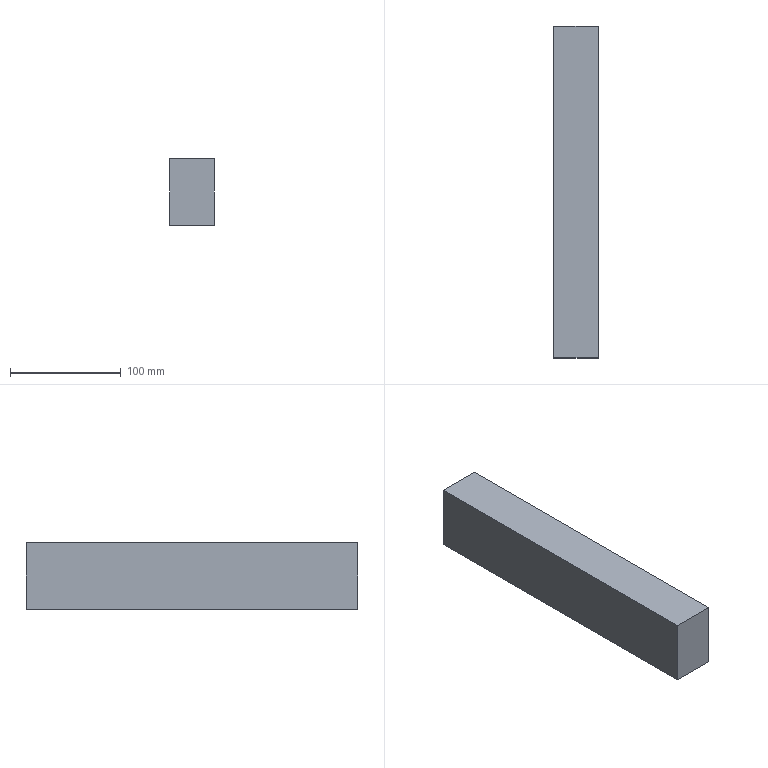Component | SolidWorks | Telescopic3-1 | 1 solid | 6 faces | box 40 x 300 x 60 mm | volume 720000 mm3 | plane 6
build123d program:
from build123d import *

# Parameters (mm, degrees)
SKETCH1_W           = 60
SKETCH1_H           = 40
BOSS_EXTRUDE1_DEPTH = 300


with BuildPart() as part:
    # Sketch1 → Boss-Extrude1 (new body)
    with BuildSketch(Plane.XY):
        Rectangle(SKETCH1_W, SKETCH1_H)
    extrude(amount=BOSS_EXTRUDE1_DEPTH)


solid = part.part

# Placed as in the assembly
solid = solid.moved(Location((-234.371, -906.787, 102.31), (90, 0, 90)))
STEP:
#1=COLOUR_RGB('',0.7922,0.8196,0.9333);
#2=FILL_AREA_STYLE_COLOUR('',#1);
#3=FILL_AREA_STYLE('',(#2));
#4=SURFACE_STYLE_FILL_AREA(#3);
#5=SURFACE_SIDE_STYLE('',(#4));
#6=SURFACE_STYLE_USAGE(.BOTH.,#5);
#7=PRESENTATION_STYLE_ASSIGNMENT((#6));
#8=CARTESIAN_POINT('',(-10.015,-47.511,5.209));
#9=VERTEX_POINT('',#8);
#10=CARTESIAN_POINT('',(-8.44,-47.511,5.209));
#11=VERTEX_POINT('',#10);
#12=CARTESIAN_POINT('',(-10.015,-47.511,5.209));
#13=DIRECTION('',(1.,-0.,-0.));
#14=VECTOR('',#13,39.37);
#15=LINE('',#12,#14);
#16=EDGE_CURVE('',#9,#11,#15,.T.);
#17=ORIENTED_EDGE('',*,*,#16,.T.);
#18=CARTESIAN_POINT('',(-8.44,-35.7,5.209));
#19=VERTEX_POINT('',#18);
#20=CARTESIAN_POINT('',(-8.44,-35.7,5.209));
#21=DIRECTION('',(-0.,-1.,0.));
#22=VECTOR('',#21,39.37);
#23=LINE('',#20,#22);
#24=EDGE_CURVE('',#19,#11,#23,.T.);
#25=ORIENTED_EDGE('',*,*,#24,.F.);
#26=CARTESIAN_POINT('',(-10.015,-35.7,5.209));
#27=VERTEX_POINT('',#26);
#28=CARTESIAN_POINT('',(-10.015,-35.7,5.209));
#29=DIRECTION('',(1.,-0.,-0.));
#30=VECTOR('',#29,39.37);
#31=LINE('',#28,#30);
#32=EDGE_CURVE('',#27,#19,#31,.T.);
#33=ORIENTED_EDGE('',*,*,#32,.F.);
#34=CARTESIAN_POINT('',(-10.015,-35.7,5.209));
#35=DIRECTION('',(-0.,-1.,0.));
#36=VECTOR('',#35,39.37);
#37=LINE('',#34,#36);
#38=EDGE_CURVE('',#27,#9,#37,.T.);
#39=ORIENTED_EDGE('',*,*,#38,.T.);
#40=EDGE_LOOP('',(#17,#25,#33,#39));
#41=FACE_OUTER_BOUND('',#40,.T.);
#42=CARTESIAN_POINT('',(-10.015,-35.7,5.209));
#43=DIRECTION('',(-0.,-0.,-1.));
#44=DIRECTION('',(0.,1.,-0.));
#45=AXIS2_PLACEMENT_3D('',#42,#43,#44);
#46=PLANE('',#45);
#47=ADVANCED_FACE('',(#41),#46,.F.);
#48=CARTESIAN_POINT('',(-8.44,-47.511,2.847));
#49=VERTEX_POINT('',#48);
#50=CARTESIAN_POINT('',(-8.44,-47.511,2.847));
#51=DIRECTION('',(-0.,-0.,-1.));
#52=VECTOR('',#51,39.37);
#53=LINE('',#50,#52);
#54=EDGE_CURVE('',#11,#49,#53,.T.);
#55=ORIENTED_EDGE('',*,*,#54,.T.);
#56=CARTESIAN_POINT('',(-8.44,-35.7,2.847));
#57=VERTEX_POINT('',#56);
#58=CARTESIAN_POINT('',(-8.44,-35.7,2.847));
#59=DIRECTION('',(-0.,-1.,0.));
#60=VECTOR('',#59,39.37);
#61=LINE('',#58,#60);
#62=EDGE_CURVE('',#57,#49,#61,.T.);
#63=ORIENTED_EDGE('',*,*,#62,.F.);
#64=CARTESIAN_POINT('',(-8.44,-35.7,2.847));
#65=DIRECTION('',(-0.,-0.,-1.));
#66=VECTOR('',#65,39.37);
#67=LINE('',#64,#66);
#68=EDGE_CURVE('',#19,#57,#67,.T.);
#69=ORIENTED_EDGE('',*,*,#68,.F.);
#70=ORIENTED_EDGE('',*,*,#24,.T.);
#71=EDGE_LOOP('',(#55,#63,#69,#70));
#72=FACE_OUTER_BOUND('',#71,.T.);
#73=CARTESIAN_POINT('',(-8.44,-35.7,2.847));
#74=DIRECTION('',(-1.,0.,0.));
#75=DIRECTION('',(-0.,-1.,0.));
#76=AXIS2_PLACEMENT_3D('',#73,#74,#75);
#77=PLANE('',#76);
#78=ADVANCED_FACE('',(#72),#77,.F.);
#79=CARTESIAN_POINT('',(-10.015,-47.511,2.847));
#80=VERTEX_POINT('',#79);
#81=CARTESIAN_POINT('',(-10.015,-47.511,2.847));
#82=DIRECTION('',(-1.,0.,0.));
#83=VECTOR('',#82,39.37);
#84=LINE('',#81,#83);
#85=EDGE_CURVE('',#49,#80,#84,.T.);
#86=ORIENTED_EDGE('',*,*,#85,.T.);
#87=CARTESIAN_POINT('',(-10.015,-35.7,2.847));
#88=VERTEX_POINT('',#87);
#89=CARTESIAN_POINT('',(-10.015,-35.7,2.847));
#90=DIRECTION('',(-0.,-1.,0.));
#91=VECTOR('',#90,39.37);
#92=LINE('',#89,#91);
#93=EDGE_CURVE('',#88,#80,#92,.T.);
#94=ORIENTED_EDGE('',*,*,#93,.F.);
#95=CARTESIAN_POINT('',(-10.015,-35.7,2.847));
#96=DIRECTION('',(-1.,0.,0.));
#97=VECTOR('',#96,39.37);
#98=LINE('',#95,#97);
#99=EDGE_CURVE('',#57,#88,#98,.T.);
#100=ORIENTED_EDGE('',*,*,#99,.F.);
#101=ORIENTED_EDGE('',*,*,#62,.T.);
#102=EDGE_LOOP('',(#86,#94,#100,#101));
#103=FACE_OUTER_BOUND('',#102,.T.);
#104=CARTESIAN_POINT('',(-10.015,-35.7,2.847));
#105=DIRECTION('',(0.,0.,1.));
#106=DIRECTION('',(-0.,-1.,0.));
#107=AXIS2_PLACEMENT_3D('',#104,#105,#106);
#108=PLANE('',#107);
#109=ADVANCED_FACE('',(#103),#108,.F.);
#110=CARTESIAN_POINT('',(-10.015,-47.511,2.847));
#111=DIRECTION('',(0.,0.,1.));
#112=VECTOR('',#111,39.37);
#113=LINE('',#110,#112);
#114=EDGE_CURVE('',#80,#9,#113,.T.);
#115=ORIENTED_EDGE('',*,*,#114,.T.);
#116=ORIENTED_EDGE('',*,*,#38,.F.);
#117=CARTESIAN_POINT('',(-10.015,-35.7,2.847));
#118=DIRECTION('',(0.,0.,1.));
#119=VECTOR('',#118,39.37);
#120=LINE('',#117,#119);
#121=EDGE_CURVE('',#88,#27,#120,.T.);
#122=ORIENTED_EDGE('',*,*,#121,.F.);
#123=ORIENTED_EDGE('',*,*,#93,.T.);
#124=EDGE_LOOP('',(#115,#116,#122,#123));
#125=FACE_OUTER_BOUND('',#124,.T.);
#126=CARTESIAN_POINT('',(-10.015,-35.7,2.847));
#127=DIRECTION('',(1.,-0.,-0.));
#128=DIRECTION('',(0.,1.,-0.));
#129=AXIS2_PLACEMENT_3D('',#126,#127,#128);
#130=PLANE('',#129);
#131=ADVANCED_FACE('',(#125),#130,.F.);
#132=ORIENTED_EDGE('',*,*,#32,.T.);
#133=ORIENTED_EDGE('',*,*,#68,.T.);
#134=ORIENTED_EDGE('',*,*,#99,.T.);
#135=ORIENTED_EDGE('',*,*,#121,.T.);
#136=EDGE_LOOP('',(#132,#133,#134,#135));
#137=FACE_OUTER_BOUND('',#136,.T.);
#138=CARTESIAN_POINT('',(-9.227,-35.7,4.028));
#139=DIRECTION('',(-0.,-1.,0.));
#140=DIRECTION('',(-0.,-0.,-1.));
#141=AXIS2_PLACEMENT_3D('',#138,#139,#140);
#142=PLANE('',#141);
#143=ADVANCED_FACE('',(#137),#142,.F.);
#144=ORIENTED_EDGE('',*,*,#16,.F.);
#145=ORIENTED_EDGE('',*,*,#114,.F.);
#146=ORIENTED_EDGE('',*,*,#85,.F.);
#147=ORIENTED_EDGE('',*,*,#54,.F.);
#148=EDGE_LOOP('',(#144,#145,#146,#147));
#149=FACE_OUTER_BOUND('',#148,.T.);
#150=CARTESIAN_POINT('',(-9.227,-47.511,4.028));
#151=DIRECTION('',(-0.,-1.,0.));
#152=DIRECTION('',(-0.,-0.,-1.));
#153=AXIS2_PLACEMENT_3D('',#150,#151,#152);
#154=PLANE('',#153);
#155=ADVANCED_FACE('',(#149),#154,.T.);
#156=CLOSED_SHELL('',(#47,#78,#109,#131,#143,#155));
#157=MANIFOLD_SOLID_BREP('',#156);
#158=STYLED_ITEM('',(#7),#157);
#159=(LENGTH_UNIT()NAMED_UNIT(*)SI_UNIT($,.METRE.));
#160=LENGTH_MEASURE_WITH_UNIT(LENGTH_MEASURE(0.0254),#159);
#161=DIMENSIONAL_EXPONENTS(1.,0.,0.,0.,0.,0.,0.);
#162=(CONVERSION_BASED_UNIT('',#160)LENGTH_UNIT()NAMED_UNIT(#161));
#163=UNCERTAINTY_MEASURE_WITH_UNIT(LENGTH_MEASURE(0.00001),#162,'','');
#164=(NAMED_UNIT(*)PLANE_ANGLE_UNIT()SI_UNIT($,.RADIAN.));
#165=(NAMED_UNIT(*)SI_UNIT($,.STERADIAN.)SOLID_ANGLE_UNIT());
#166=(GEOMETRIC_REPRESENTATION_CONTEXT(3)GLOBAL_UNCERTAINTY_ASSIGNED_CONTEXT((#163))GLOBAL_UNIT_ASSIGNED_CONTEXT((#162,#164,#165))REPRESENTATION_CONTEXT('',''));
#167=MECHANICAL_DESIGN_GEOMETRIC_PRESENTATION_REPRESENTATION('',(#158),#166);
#168=PRESENTATION_LAYER_ASSIGNMENT('','',(#158));
#169=CARTESIAN_POINT('',(0.,0.,0.));
#170=DIRECTION('',(0.,0.,1.));
#171=DIRECTION('',(1.,0.,0.));
#172=AXIS2_PLACEMENT_3D('',#169,#170,#171);
#173=(LENGTH_UNIT()NAMED_UNIT(*)SI_UNIT($,.METRE.));
#174=LENGTH_MEASURE_WITH_UNIT(LENGTH_MEASURE(0.0254),#173);
#175=DIMENSIONAL_EXPONENTS(1.,0.,0.,0.,0.,0.,0.);
#176=(CONVERSION_BASED_UNIT('',#174)LENGTH_UNIT()NAMED_UNIT(#175));
#177=UNCERTAINTY_MEASURE_WITH_UNIT(LENGTH_MEASURE(0.00001),#176,'','');
#178=(NAMED_UNIT(*)PLANE_ANGLE_UNIT()SI_UNIT($,.RADIAN.));
#179=(NAMED_UNIT(*)SI_UNIT($,.STERADIAN.)SOLID_ANGLE_UNIT());
#180=(GEOMETRIC_REPRESENTATION_CONTEXT(3)GLOBAL_UNCERTAINTY_ASSIGNED_CONTEXT((#177))GLOBAL_UNIT_ASSIGNED_CONTEXT((#176,#178,#179))REPRESENTATION_CONTEXT('',''));
#181=ADVANCED_BREP_SHAPE_REPRESENTATION('',(#157,#172),#180);